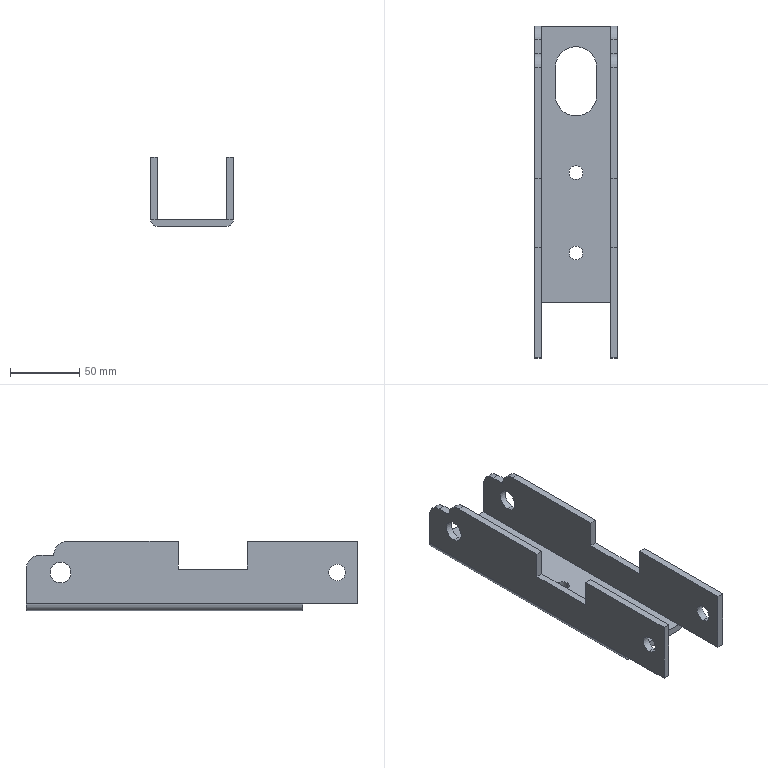Component | SolidWorks | SeederFixingFrame-1 | 1 solid | 46 faces | volume 143207 mm3 | plane 26 | cylinder 20 | commonest cylinder face diameters 10 x6 15 x4 12 x4 20 x4 30 x2